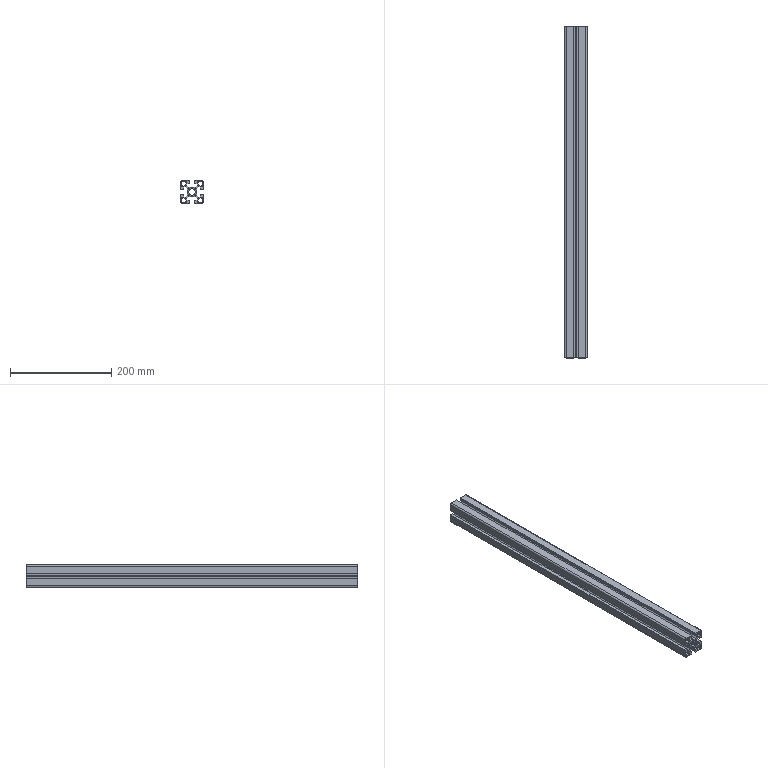Component | SolidWorks | HFS8_4545_05-B-1 | 1 solid | 131 faces | box 45 x 655 x 45 mm | volume 525441 mm3 | plane 82 | cylinder 49 | commonest cylinder face diameters 2 x18 3 x12 1 x10 12.5 x5 6 x4
build123d program:
from build123d import *

# Parameters (mm, degrees)
BOSS_EXTRUDE1_DEPTH = 655


with BuildPart() as part:
    # Sketch1 → Boss-Extrude1 (new body)
    with BuildSketch(Plane.XY):
        with BuildLine():
            Line((-19.5, -22.5), (-5, -22.5))
            Line((-5, -22.5), (-5, -16.5))
            Line((-5, -16.5), (-10, -16.5))
            Line((-10, -16.5), (-10, -13))
            Line((-10, -13), (-6.5, -9.5))
            Line((-6.5, -9.5), (-1.212, -9.5))
            Line((-1.212, -9.5), (0, -8.8))
            Line((0, -8.8), (1.212, -9.5))
            Line((1.212, -9.5), (6.5, -9.5))
            Line((6.5, -9.5), (10, -13))
            Line((10, -13), (10, -16.5))
            Line((10, -16.5), (5, -16.5))
            Line((5, -16.5), (5, -22.5))
            Line((5, -22.5), (19.5, -22.5))
            ThreePointArc((19.5, -22.5), (21.621, -21.621), (22.5, -19.5))
            Line((22.5, -19.5), (22.5, -5))
            Line((22.5, -5), (16.5, -5))
            Line((16.5, -5), (16.5, -10))
            Line((16.5, -10), (13, -10))
            Line((13, -10), (9.5, -6.5))
            Line((9.5, -6.5), (9.5, -1.212))
            Line((9.5, -1.212), (8.8, 0))
            Line((8.8, 0), (9.5, 1.212))
            Line((9.5, 1.212), (9.5, 6.5))
            Line((9.5, 6.5), (13, 10))
            Line((13, 10), (16.5, 10))
            Line((16.5, 10), (16.5, 5))
            Line((16.5, 5), (22.5, 5))
            Line((22.5, 5), (22.5, 19.5))
            ThreePointArc((22.5, 19.5), (21.621, 21.621), (19.5, 22.5))
            Line((19.5, 22.5), (5, 22.5))
            Line((5, 22.5), (5, 16.5))
            Line((5, 16.5), (10, 16.5))
            Line((10, 16.5), (10, 13))
            Line((10, 13), (6.5, 9.5))
            Line((6.5, 9.5), (1.212, 9.5))
            Line((1.212, 9.5), (0, 8.8))
            Line((0, 8.8), (-1.212, 9.5))
            Line((-1.212, 9.5), (-6.5, 9.5))
            Line((-6.5, 9.5), (-10, 13))
            Line((-10, 13), (-10, 16.5))
            Line((-10, 16.5), (-5, 16.5))
            Line((-5, 16.5), (-5, 22.5))
            Line((-5, 22.5), (-19.5, 22.5))
            ThreePointArc((-19.5, 22.5), (-21.621, 21.621), (-22.5, 19.5))
            Line((-22.5, 19.5), (-22.5, 5))
            Line((-22.5, 5), (-16.5, 5))
            Line((-16.5, 5), (-16.5, 10))
            Line((-16.5, 10), (-13, 10))
            Line((-13, 10), (-9.5, 6.5))
            Line((-9.5, 6.5), (-9.5, 1.212))
            Line((-9.5, 1.212), (-8.8, 0))
            Line((-8.8, 0), (-9.5, -1.212))
            Line((-9.5, -1.212), (-9.5, -6.5))
            Line((-9.5, -6.5), (-13, -10))
            Line((-13, -10), (-16.5, -10))
            Line((-16.5, -10), (-16.5, -5))
            Line((-16.5, -5), (-22.5, -5))
            Line((-22.5, -5), (-22.5, -19.5))
            ThreePointArc((-22.5, -19.5), (-21.621, -21.621), (-19.5, -22.5))
        make_face()
        with BuildLine():
            Line((12, 18.5), (12, 13))
            ThreePointArc((12, 13), (12.293, 12.293), (13, 12))
            Line((13, 12), (18.5, 12))
            ThreePointArc((18.5, 12), (19.5, 11), (20.5, 12))
            Line((20.5, 12), (20.5, 19.5))
            ThreePointArc((20.5, 19.5), (20.207, 20.207), (19.5, 20.5))
            Line((19.5, 20.5), (12, 20.5))
            ThreePointArc((12, 20.5), (11, 19.5), (12, 18.5))
        make_face(mode=Mode.SUBTRACT)
        with BuildLine():
            Line((12, -20.5), (19.5, -20.5))
            ThreePointArc((19.5, -20.5), (20.207, -20.207), (20.5, -19.5))
            Line((20.5, -19.5), (20.5, -12))
            ThreePointArc((20.5, -12), (19.5, -11), (18.5, -12))
            Line((18.5, -12), (13, -12))
            ThreePointArc((13, -12), (12.293, -12.293), (12, -13))
            Line((12, -13), (12, -18.5))
            ThreePointArc((12, -18.5), (11, -19.5), (12, -20.5))
        make_face(mode=Mode.SUBTRACT)
        with BuildLine():
            Line((-4.725, -6.139), (-3.947, -5.361))
            ThreePointArc((-3.947, -5.361), (-3.649, -5.217), (-3.327, -5.291))
            ThreePointArc((-3.327, -5.291), (0, -6.25), (3.327, -5.291))
            ThreePointArc((3.327, -5.291), (3.649, -5.217), (3.947, -5.361))
            Line((3.947, -5.361), (4.725, -6.139))
            ThreePointArc((4.725, -6.139), (7.283, -7.283), (6.139, -4.725))
            Line((6.139, -4.725), (5.361, -3.947))
            ThreePointArc((5.361, -3.947), (5.217, -3.649), (5.291, -3.327))
            ThreePointArc((5.291, -3.327), (6.25, 0), (5.291, 3.327))
            ThreePointArc((5.291, 3.327), (5.217, 3.649), (5.361, 3.947))
            Line((5.361, 3.947), (6.139, 4.725))
            ThreePointArc((6.139, 4.725), (7.283, 7.283), (4.725, 6.139))
            Line((4.725, 6.139), (3.947, 5.361))
            ThreePointArc((3.947, 5.361), (3.649, 5.217), (3.327, 5.291))
            ThreePointArc((3.327, 5.291), (0, 6.25), (-3.327, 5.291))
            ThreePointArc((-3.327, 5.291), (-3.649, 5.217), (-3.947, 5.361))
            Line((-3.947, 5.361), (-4.725, 6.139))
            ThreePointArc((-4.725, 6.139), (-7.283, 7.283), (-6.139, 4.725))
            Line((-6.139, 4.725), (-5.361, 3.947))
            ThreePointArc((-5.361, 3.947), (-5.217, 3.649), (-5.291, 3.327))
            ThreePointArc((-5.291, 3.327), (-6.25, 0), (-5.291, -3.327))
            ThreePointArc((-5.291, -3.327), (-5.217, -3.649), (-5.361, -3.947))
            Line((-5.361, -3.947), (-6.139, -4.725))
            ThreePointArc((-6.139, -4.725), (-7.283, -7.283), (-4.725, -6.139))
        make_face(mode=Mode.SUBTRACT)
        with BuildLine():
            Line((-19.5, -20.5), (-12, -20.5))
            ThreePointArc((-12, -20.5), (-11, -19.5), (-12, -18.5))
            Line((-12, -18.5), (-12, -13))
            ThreePointArc((-12, -13), (-12.293, -12.293), (-13, -12))
            Line((-13, -12), (-18.5, -12))
            ThreePointArc((-18.5, -12), (-19.5, -11), (-20.5, -12))
            Line((-20.5, -12), (-20.5, -19.5))
            ThreePointArc((-20.5, -19.5), (-20.207, -20.207), (-19.5, -20.5))
        make_face(mode=Mode.SUBTRACT)
        with BuildLine():
            Line((-18.5, 12), (-13, 12))
            ThreePointArc((-13, 12), (-12.293, 12.293), (-12, 13))
            Line((-12, 13), (-12, 18.5))
            ThreePointArc((-12, 18.5), (-11, 19.5), (-12, 20.5))
            Line((-12, 20.5), (-19.5, 20.5))
            ThreePointArc((-19.5, 20.5), (-20.207, 20.207), (-20.5, 19.5))
            Line((-20.5, 19.5), (-20.5, 12))
            ThreePointArc((-20.5, 12), (-19.5, 11), (-18.5, 12))
        make_face(mode=Mode.SUBTRACT)
    extrude(amount=-BOSS_EXTRUDE1_DEPTH)


solid = part.part

# Placed as in the assembly
solid = solid.moved(Location((-65.506, -669.413, -2380.428), (90, 0, 0)))